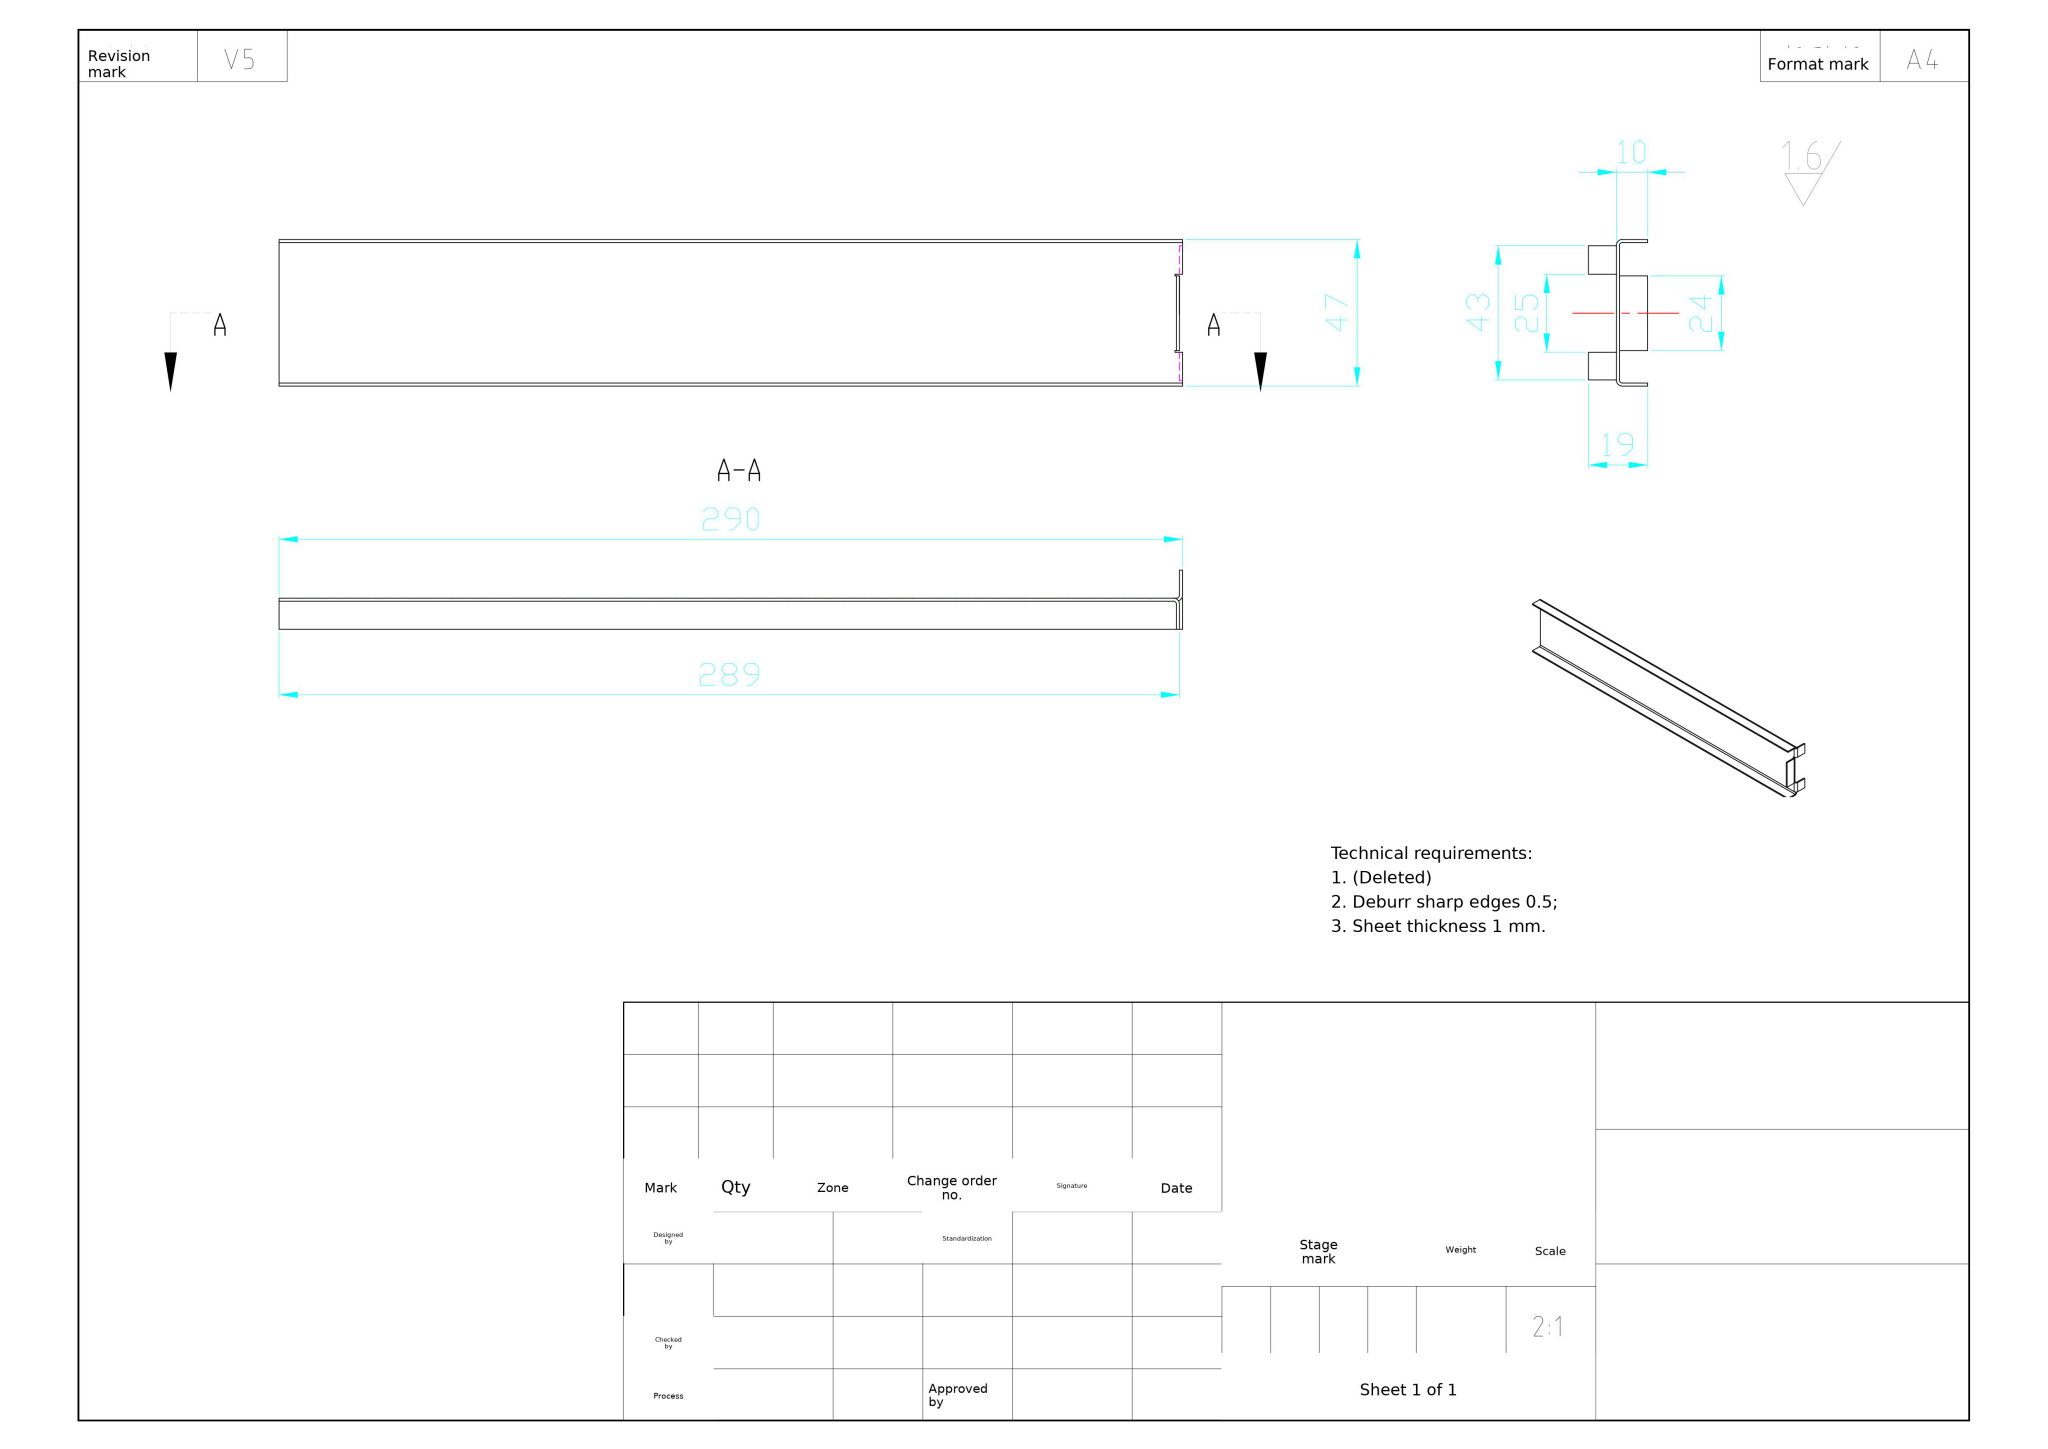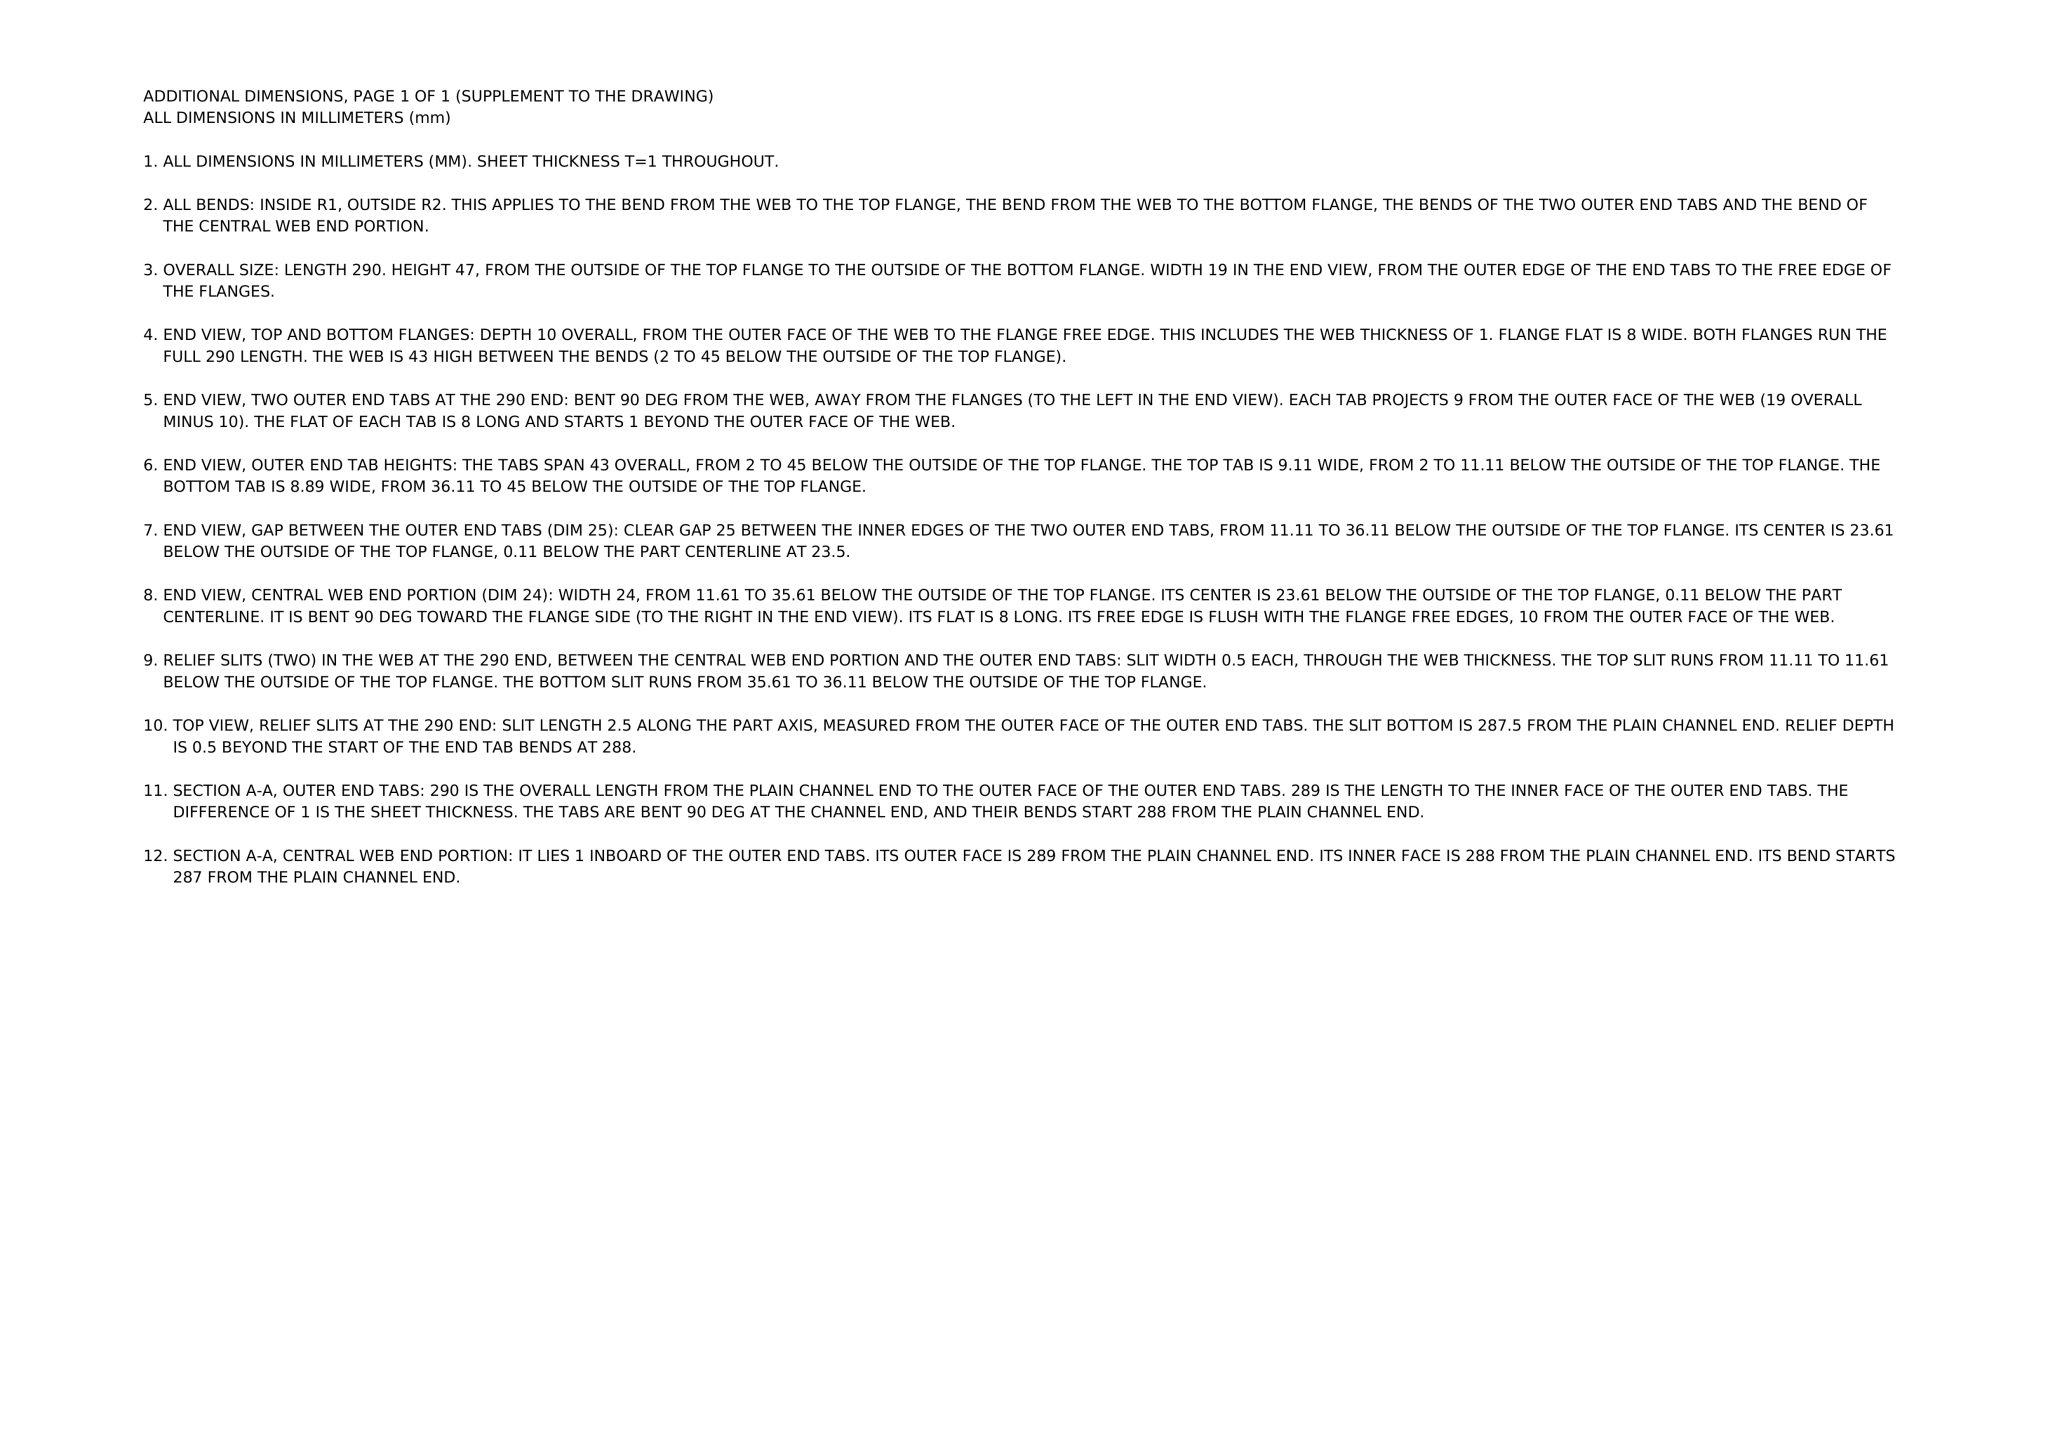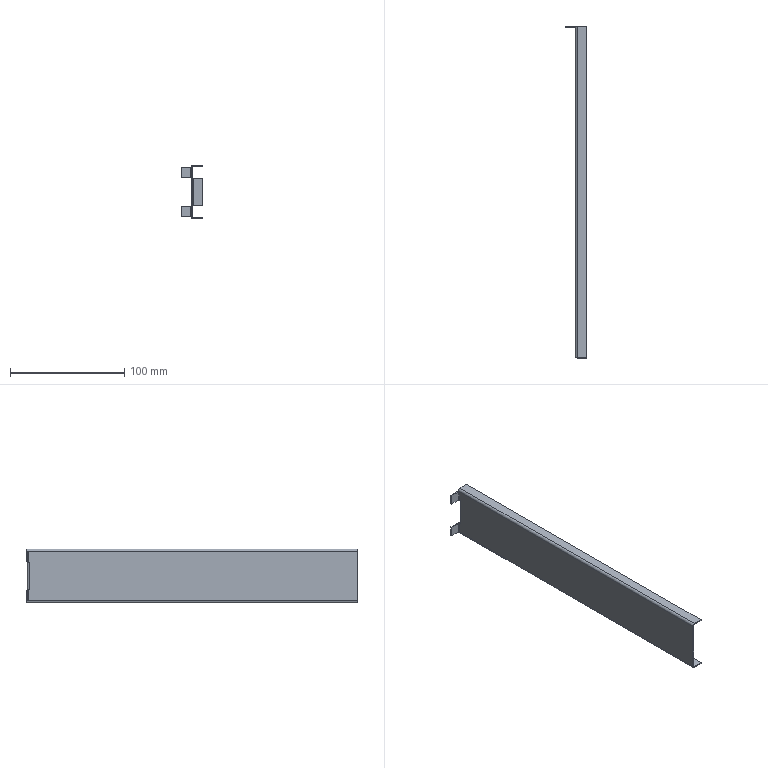Part | NX | mm | 1 solid | 56 faces | box 19 x 290 x 47 mm | volume 18801 mm3 | plane 46 | cylinder 10 | commonest cylinder face diameters 4 x5 2 x5